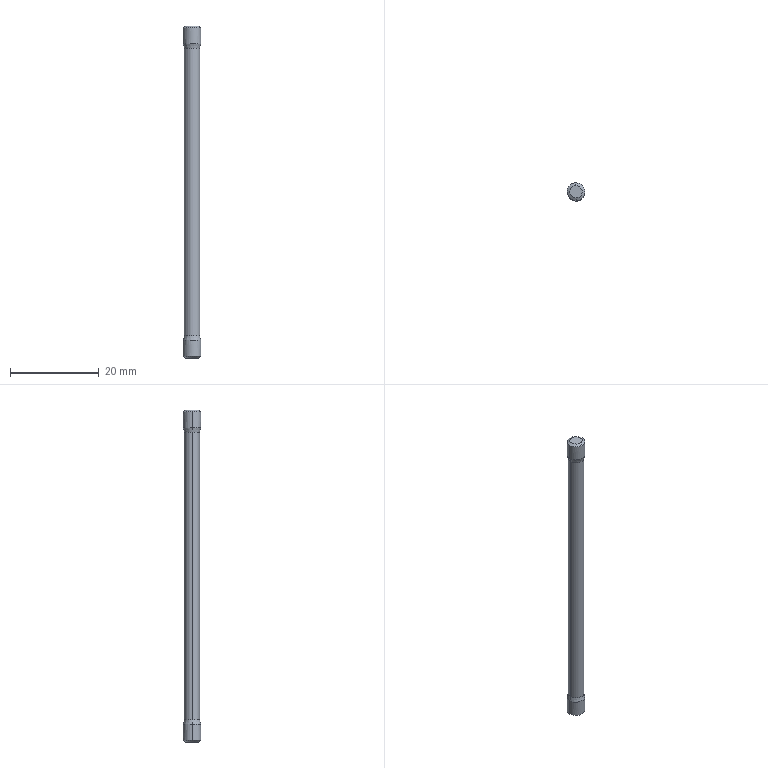Component | SolidWorks | GB_T901-1988EqualLengthDoubleEndStudGradeBM4x75-1 | 1 solid | 16 faces | box 4 x 4 x 75 mm | volume 733 mm3 | cone 8 | cylinder 6 | plane 2 | commonest cylinder face diameters 4 x4 3.464 x2
build123d program:
from build123d import *


with BuildPart() as part:
    # Sketch1 → Base-Revolve (revolve)
    with BuildSketch(Plane.XY, mode=Mode.PRIVATE) as base_revolve_sk:
        Polygon((-37.5, 2), (-33.5, 2), (-32.52, 1.732), (0, 1.732), (0, 0), (-37.5, 0), align=None)
    revolve(base_revolve_sk.sketch.rotate(Axis((-37.5, 0, 0), (1, 0, 0)), 180), axis=Axis((-37.5, 0, 0), (1, 0, 0)))

    # Sketch2 → Thread Cut (revolve, cut)
    with BuildSketch(Plane.XY, mode=Mode.PRIVATE) as thread_cut_sk:
        Polygon((-37.85, 2), (-37.15, 2), (-37.5, 1.394), align=None)
    revolve(thread_cut_sk.sketch.rotate(Axis((-26.952, 0, 0), (1, 0, 0)), 180), axis=Axis((-26.952, 0, 0), (1, 0, 0)), mode=Mode.SUBTRACT)

    # Mirror All1: part across plane


with BuildPart() as part_1:
    add(part.part)
    add(part.part.mirror(Plane(origin=(0, 1.732, 0), x_dir=(0, 0, 1), z_dir=(-1, 0, 0))))


solid = part_1.part

# Placed as in the assembly
solid = solid.moved(Location((18.125, -13.646, 22.463), (0, 90, 0)))
STEP:
#1=CARTESIAN_POINT('',(0.7155,-0.5921,2.361));
#2=VERTEX_POINT('',#1);
#3=CARTESIAN_POINT('',(0.7117,-0.4824,2.361));
#4=VERTEX_POINT('',#3);
#5=CARTESIAN_POINT('',(0.7136,-0.5373,2.361));
#6=DIRECTION('',(0.,0.,-1.));
#7=DIRECTION('',(-0.0348,0.9994,0.));
#8=AXIS2_PLACEMENT_3D('',#5,#6,#7);
#9=CIRCLE('',#8,0.05487);
#10=EDGE_CURVE('',#2,#4,#9,.T.);
#11=ORIENTED_EDGE('',*,*,#10,.T.);
#12=CARTESIAN_POINT('',(0.7108,-0.4586,2.347));
#13=VERTEX_POINT('',#12);
#14=CARTESIAN_POINT('',(0.7117,-0.4824,2.361));
#15=DIRECTION('',(-0.03014,0.8655,-0.5));
#16=VECTOR('',#15,39.37);
#17=LINE('',#14,#16);
#18=EDGE_CURVE('',#4,#13,#17,.T.);
#19=ORIENTED_EDGE('',*,*,#18,.T.);
#20=CARTESIAN_POINT('',(0.6349,-0.54,2.347));
#21=VERTEX_POINT('',#20);
#22=CARTESIAN_POINT('',(0.7136,-0.5373,2.347));
#23=DIRECTION('',(0.,0.,-1.));
#24=DIRECTION('',(-0.0348,0.9994,0.));
#25=AXIS2_PLACEMENT_3D('',#22,#23,#24);
#26=CIRCLE('',#25,0.07874);
#27=EDGE_CURVE('',#21,#13,#26,.T.);
#28=ORIENTED_EDGE('',*,*,#27,.F.);
#29=CARTESIAN_POINT('',(0.7163,-0.616,2.347));
#30=VERTEX_POINT('',#29);
#31=CARTESIAN_POINT('',(0.7136,-0.5373,2.347));
#32=DIRECTION('',(0.,0.,-1.));
#33=DIRECTION('',(-0.0348,0.9994,0.));
#34=AXIS2_PLACEMENT_3D('',#31,#32,#33);
#35=CIRCLE('',#34,0.07874);
#36=EDGE_CURVE('',#30,#21,#35,.T.);
#37=ORIENTED_EDGE('',*,*,#36,.F.);
#38=CARTESIAN_POINT('',(0.7155,-0.5921,2.361));
#39=DIRECTION('',(0.03014,-0.8655,-0.5));
#40=VECTOR('',#39,39.37);
#41=LINE('',#38,#40);
#42=EDGE_CURVE('',#2,#30,#41,.T.);
#43=ORIENTED_EDGE('',*,*,#42,.F.);
#44=EDGE_LOOP('',(#11,#19,#28,#37,#43));
#45=FACE_OUTER_BOUND('',#44,.T.);
#46=CARTESIAN_POINT('',(0.7136,-0.5373,2.361));
#47=DIRECTION('',(0.,0.,-1.));
#48=DIRECTION('',(0.0348,-0.9994,0.));
#49=AXIS2_PLACEMENT_3D('',#46,#47,#48);
#50=CONICAL_SURFACE('',#49,0.05487,1.047);
#51=ADVANCED_FACE('',(#45),#50,.T.);
#52=CARTESIAN_POINT('',(0.7817,-0.5349,2.165));
#53=VERTEX_POINT('',#52);
#54=CARTESIAN_POINT('',(0.6454,-0.5396,2.165));
#55=VERTEX_POINT('',#54);
#56=CARTESIAN_POINT('',(0.7136,-0.5373,2.165));
#57=DIRECTION('',(0.,0.,-1.));
#58=DIRECTION('',(-0.9994,-0.0348,0.));
#59=AXIS2_PLACEMENT_3D('',#56,#57,#58);
#60=CIRCLE('',#59,0.06819);
#61=EDGE_CURVE('',#53,#55,#60,.T.);
#62=ORIENTED_EDGE('',*,*,#61,.F.);
#63=CARTESIAN_POINT('',(0.7923,-0.5345,2.203));
#64=VERTEX_POINT('',#63);
#65=CARTESIAN_POINT('',(0.7817,-0.5349,2.165));
#66=DIRECTION('',(0.2636,0.00918,0.9646));
#67=VECTOR('',#66,39.37);
#68=LINE('',#65,#67);
#69=EDGE_CURVE('',#53,#64,#68,.T.);
#70=ORIENTED_EDGE('',*,*,#69,.T.);
#71=CARTESIAN_POINT('',(0.6349,-0.54,2.203));
#72=VERTEX_POINT('',#71);
#73=CARTESIAN_POINT('',(0.7136,-0.5373,2.203));
#74=DIRECTION('',(0.,0.,-1.));
#75=DIRECTION('',(-0.9994,-0.0348,0.));
#76=AXIS2_PLACEMENT_3D('',#73,#74,#75);
#77=CIRCLE('',#76,0.07874);
#78=EDGE_CURVE('',#64,#72,#77,.T.);
#79=ORIENTED_EDGE('',*,*,#78,.T.);
#80=CARTESIAN_POINT('',(0.6454,-0.5396,2.165));
#81=DIRECTION('',(-0.2636,-0.00918,0.9646));
#82=VECTOR('',#81,39.37);
#83=LINE('',#80,#82);
#84=EDGE_CURVE('',#55,#72,#83,.T.);
#85=ORIENTED_EDGE('',*,*,#84,.F.);
#86=EDGE_LOOP('',(#62,#70,#79,#85));
#87=FACE_OUTER_BOUND('',#86,.T.);
#88=CARTESIAN_POINT('',(0.7136,-0.5373,2.165));
#89=DIRECTION('',(-0.,-0.,1.));
#90=DIRECTION('',(-0.9994,-0.0348,0.));
#91=AXIS2_PLACEMENT_3D('',#88,#89,#90);
#92=CONICAL_SURFACE('',#91,0.06819,0.2669);
#93=ADVANCED_FACE('',(#87),#92,.T.);
#94=ORIENTED_EDGE('',*,*,#78,.F.);
#95=CARTESIAN_POINT('',(0.7923,-0.5345,2.347));
#96=VERTEX_POINT('',#95);
#97=CARTESIAN_POINT('',(0.7923,-0.5345,2.361));
#98=DIRECTION('',(-0.,-0.,1.));
#99=VECTOR('',#98,39.37);
#100=LINE('',#97,#99);
#101=EDGE_CURVE('',#64,#96,#100,.T.);
#102=ORIENTED_EDGE('',*,*,#101,.T.);
#103=CARTESIAN_POINT('',(0.7136,-0.5373,2.347));
#104=DIRECTION('',(0.,0.,-1.));
#105=DIRECTION('',(-0.0348,0.9994,0.));
#106=AXIS2_PLACEMENT_3D('',#103,#104,#105);
#107=CIRCLE('',#106,0.07874);
#108=EDGE_CURVE('',#96,#30,#107,.T.);
#109=ORIENTED_EDGE('',*,*,#108,.T.);
#110=ORIENTED_EDGE('',*,*,#36,.T.);
#111=CARTESIAN_POINT('',(0.6349,-0.54,2.361));
#112=DIRECTION('',(-0.,-0.,1.));
#113=VECTOR('',#112,39.37);
#114=LINE('',#111,#113);
#115=EDGE_CURVE('',#72,#21,#114,.T.);
#116=ORIENTED_EDGE('',*,*,#115,.F.);
#117=EDGE_LOOP('',(#94,#102,#109,#110,#116));
#118=FACE_OUTER_BOUND('',#117,.T.);
#119=CARTESIAN_POINT('',(0.7136,-0.5373,2.361));
#120=DIRECTION('',(-0.,-0.,1.));
#121=DIRECTION('',(-0.9994,-0.0348,0.));
#122=AXIS2_PLACEMENT_3D('',#119,#120,#121);
#123=CYLINDRICAL_SURFACE('',#122,0.07874);
#124=ADVANCED_FACE('',(#118),#123,.T.);
#125=CARTESIAN_POINT('',(0.7117,-0.4824,-0.592));
#126=VERTEX_POINT('',#125);
#127=CARTESIAN_POINT('',(0.7155,-0.5921,-0.592));
#128=VERTEX_POINT('',#127);
#129=CARTESIAN_POINT('',(0.7136,-0.5373,-0.592));
#130=DIRECTION('',(0.,0.,-1.));
#131=DIRECTION('',(-0.0348,0.9994,0.));
#132=AXIS2_PLACEMENT_3D('',#129,#130,#131);
#133=CIRCLE('',#132,0.05487);
#134=EDGE_CURVE('',#126,#128,#133,.T.);
#135=ORIENTED_EDGE('',*,*,#134,.F.);
#136=CARTESIAN_POINT('',(0.7108,-0.4586,-0.5782));
#137=VERTEX_POINT('',#136);
#138=CARTESIAN_POINT('',(0.7117,-0.4824,-0.592));
#139=DIRECTION('',(-0.03014,0.8655,0.5));
#140=VECTOR('',#139,39.37);
#141=LINE('',#138,#140);
#142=EDGE_CURVE('',#126,#137,#141,.T.);
#143=ORIENTED_EDGE('',*,*,#142,.T.);
#144=CARTESIAN_POINT('',(0.7923,-0.5345,-0.5782));
#145=VERTEX_POINT('',#144);
#146=CARTESIAN_POINT('',(0.7136,-0.5373,-0.5782));
#147=DIRECTION('',(0.,0.,-1.));
#148=DIRECTION('',(-0.0348,0.9994,0.));
#149=AXIS2_PLACEMENT_3D('',#146,#147,#148);
#150=CIRCLE('',#149,0.07874);
#151=EDGE_CURVE('',#137,#145,#150,.T.);
#152=ORIENTED_EDGE('',*,*,#151,.T.);
#153=CARTESIAN_POINT('',(0.7163,-0.616,-0.5782));
#154=VERTEX_POINT('',#153);
#155=CARTESIAN_POINT('',(0.7136,-0.5373,-0.5782));
#156=DIRECTION('',(0.,0.,-1.));
#157=DIRECTION('',(-0.0348,0.9994,0.));
#158=AXIS2_PLACEMENT_3D('',#155,#156,#157);
#159=CIRCLE('',#158,0.07874);
#160=EDGE_CURVE('',#145,#154,#159,.T.);
#161=ORIENTED_EDGE('',*,*,#160,.T.);
#162=CARTESIAN_POINT('',(0.7155,-0.5921,-0.592));
#163=DIRECTION('',(0.03014,-0.8655,0.5));
#164=VECTOR('',#163,39.37);
#165=LINE('',#162,#164);
#166=EDGE_CURVE('',#128,#154,#165,.T.);
#167=ORIENTED_EDGE('',*,*,#166,.F.);
#168=EDGE_LOOP('',(#135,#143,#152,#161,#167));
#169=FACE_OUTER_BOUND('',#168,.T.);
#170=CARTESIAN_POINT('',(0.7136,-0.5373,-0.592));
#171=DIRECTION('',(-0.,-0.,1.));
#172=DIRECTION('',(0.0348,-0.9994,0.));
#173=AXIS2_PLACEMENT_3D('',#170,#171,#172);
#174=CONICAL_SURFACE('',#173,0.05487,1.047);
#175=ADVANCED_FACE('',(#169),#174,.T.);
#176=CARTESIAN_POINT('',(0.6454,-0.5396,-0.3959));
#177=VERTEX_POINT('',#176);
#178=CARTESIAN_POINT('',(0.7817,-0.5349,-0.3959));
#179=VERTEX_POINT('',#178);
#180=CARTESIAN_POINT('',(0.7136,-0.5373,-0.3959));
#181=DIRECTION('',(0.,0.,-1.));
#182=DIRECTION('',(-0.9994,-0.0348,0.));
#183=AXIS2_PLACEMENT_3D('',#180,#181,#182);
#184=CIRCLE('',#183,0.06819);
#185=EDGE_CURVE('',#177,#179,#184,.T.);
#186=ORIENTED_EDGE('',*,*,#185,.T.);
#187=CARTESIAN_POINT('',(0.7923,-0.5345,-0.4345));
#188=VERTEX_POINT('',#187);
#189=CARTESIAN_POINT('',(0.7817,-0.5349,-0.3959));
#190=DIRECTION('',(0.2636,0.00918,-0.9646));
#191=VECTOR('',#190,39.37);
#192=LINE('',#189,#191);
#193=EDGE_CURVE('',#179,#188,#192,.T.);
#194=ORIENTED_EDGE('',*,*,#193,.T.);
#195=CARTESIAN_POINT('',(0.6349,-0.54,-0.4345));
#196=VERTEX_POINT('',#195);
#197=CARTESIAN_POINT('',(0.7136,-0.5373,-0.4345));
#198=DIRECTION('',(0.,0.,-1.));
#199=DIRECTION('',(-0.9994,-0.0348,0.));
#200=AXIS2_PLACEMENT_3D('',#197,#198,#199);
#201=CIRCLE('',#200,0.07874);
#202=EDGE_CURVE('',#196,#188,#201,.T.);
#203=ORIENTED_EDGE('',*,*,#202,.F.);
#204=CARTESIAN_POINT('',(0.6454,-0.5396,-0.3959));
#205=DIRECTION('',(-0.2636,-0.00918,-0.9646));
#206=VECTOR('',#205,39.37);
#207=LINE('',#204,#206);
#208=EDGE_CURVE('',#177,#196,#207,.T.);
#209=ORIENTED_EDGE('',*,*,#208,.F.);
#210=EDGE_LOOP('',(#186,#194,#203,#209));
#211=FACE_OUTER_BOUND('',#210,.T.);
#212=CARTESIAN_POINT('',(0.7136,-0.5373,-0.3959));
#213=DIRECTION('',(0.,0.,-1.));
#214=DIRECTION('',(-0.9994,-0.0348,0.));
#215=AXIS2_PLACEMENT_3D('',#212,#213,#214);
#216=CONICAL_SURFACE('',#215,0.06819,0.2669);
#217=ADVANCED_FACE('',(#211),#216,.T.);
#218=CARTESIAN_POINT('',(0.7136,-0.5373,2.165));
#219=DIRECTION('',(0.,0.,-1.));
#220=DIRECTION('',(-0.9994,-0.0348,0.));
#221=AXIS2_PLACEMENT_3D('',#218,#219,#220);
#222=CIRCLE('',#221,0.06819);
#223=EDGE_CURVE('',#55,#53,#222,.T.);
#224=ORIENTED_EDGE('',*,*,#223,.T.);
#225=CARTESIAN_POINT('',(0.7817,-0.5349,-0.592));
#226=DIRECTION('',(0.,0.,-1.));
#227=VECTOR('',#226,39.37);
#228=LINE('',#225,#227);
#229=EDGE_CURVE('',#53,#179,#228,.T.);
#230=ORIENTED_EDGE('',*,*,#229,.T.);
#231=ORIENTED_EDGE('',*,*,#185,.F.);
#232=CARTESIAN_POINT('',(0.6454,-0.5396,-0.592));
#233=DIRECTION('',(0.,0.,-1.));
#234=VECTOR('',#233,39.37);
#235=LINE('',#232,#234);
#236=EDGE_CURVE('',#55,#177,#235,.T.);
#237=ORIENTED_EDGE('',*,*,#236,.F.);
#238=EDGE_LOOP('',(#224,#230,#231,#237));
#239=FACE_OUTER_BOUND('',#238,.T.);
#240=CARTESIAN_POINT('',(0.7136,-0.5373,-0.592));
#241=DIRECTION('',(0.,0.,-1.));
#242=DIRECTION('',(-0.9994,-0.0348,0.));
#243=AXIS2_PLACEMENT_3D('',#240,#241,#242);
#244=CYLINDRICAL_SURFACE('',#243,0.06819);
#245=ADVANCED_FACE('',(#239),#244,.T.);
#246=ORIENTED_EDGE('',*,*,#202,.T.);
#247=CARTESIAN_POINT('',(0.7923,-0.5345,-0.592));
#248=DIRECTION('',(0.,0.,-1.));
#249=VECTOR('',#248,39.37);
#250=LINE('',#247,#249);
#251=EDGE_CURVE('',#188,#145,#250,.T.);
#252=ORIENTED_EDGE('',*,*,#251,.T.);
#253=ORIENTED_EDGE('',*,*,#151,.F.);
#254=CARTESIAN_POINT('',(0.6349,-0.54,-0.5782));
#255=VERTEX_POINT('',#254);
#256=CARTESIAN_POINT('',(0.7136,-0.5373,-0.5782));
#257=DIRECTION('',(0.,0.,-1.));
#258=DIRECTION('',(-0.0348,0.9994,0.));
#259=AXIS2_PLACEMENT_3D('',#256,#257,#258);
#260=CIRCLE('',#259,0.07874);
#261=EDGE_CURVE('',#255,#137,#260,.T.);
#262=ORIENTED_EDGE('',*,*,#261,.F.);
#263=CARTESIAN_POINT('',(0.6349,-0.54,-0.592));
#264=DIRECTION('',(0.,0.,-1.));
#265=VECTOR('',#264,39.37);
#266=LINE('',#263,#265);
#267=EDGE_CURVE('',#196,#255,#266,.T.);
#268=ORIENTED_EDGE('',*,*,#267,.F.);
#269=EDGE_LOOP('',(#246,#252,#253,#262,#268));
#270=FACE_OUTER_BOUND('',#269,.T.);
#271=CARTESIAN_POINT('',(0.7136,-0.5373,-0.592));
#272=DIRECTION('',(0.,0.,-1.));
#273=DIRECTION('',(-0.9994,-0.0348,0.));
#274=AXIS2_PLACEMENT_3D('',#271,#272,#273);
#275=CYLINDRICAL_SURFACE('',#274,0.07874);
#276=ADVANCED_FACE('',(#270),#275,.T.);
#277=ORIENTED_EDGE('',*,*,#251,.F.);
#278=CARTESIAN_POINT('',(0.7136,-0.5373,-0.4345));
#279=DIRECTION('',(0.,0.,-1.));
#280=DIRECTION('',(-0.9994,-0.0348,0.));
#281=AXIS2_PLACEMENT_3D('',#278,#279,#280);
#282=CIRCLE('',#281,0.07874);
#283=EDGE_CURVE('',#188,#196,#282,.T.);
#284=ORIENTED_EDGE('',*,*,#283,.T.);
#285=ORIENTED_EDGE('',*,*,#267,.T.);
#286=CARTESIAN_POINT('',(0.7136,-0.5373,-0.5782));
#287=DIRECTION('',(0.,0.,-1.));
#288=DIRECTION('',(-0.0348,0.9994,0.));
#289=AXIS2_PLACEMENT_3D('',#286,#287,#288);
#290=CIRCLE('',#289,0.07874);
#291=EDGE_CURVE('',#154,#255,#290,.T.);
#292=ORIENTED_EDGE('',*,*,#291,.F.);
#293=ORIENTED_EDGE('',*,*,#160,.F.);
#294=EDGE_LOOP('',(#277,#284,#285,#292,#293));
#295=FACE_OUTER_BOUND('',#294,.T.);
#296=CARTESIAN_POINT('',(0.7136,-0.5373,-0.592));
#297=DIRECTION('',(0.,0.,-1.));
#298=DIRECTION('',(-0.9994,-0.0348,0.));
#299=AXIS2_PLACEMENT_3D('',#296,#297,#298);
#300=CYLINDRICAL_SURFACE('',#299,0.07874);
#301=ADVANCED_FACE('',(#295),#300,.T.);
#302=ORIENTED_EDGE('',*,*,#229,.F.);
#303=ORIENTED_EDGE('',*,*,#61,.T.);
#304=ORIENTED_EDGE('',*,*,#236,.T.);
#305=CARTESIAN_POINT('',(0.7136,-0.5373,-0.3959));
#306=DIRECTION('',(0.,0.,-1.));
#307=DIRECTION('',(-0.9994,-0.0348,0.));
#308=AXIS2_PLACEMENT_3D('',#305,#306,#307);
#309=CIRCLE('',#308,0.06819);
#310=EDGE_CURVE('',#179,#177,#309,.T.);
#311=ORIENTED_EDGE('',*,*,#310,.F.);
#312=EDGE_LOOP('',(#302,#303,#304,#311));
#313=FACE_OUTER_BOUND('',#312,.T.);
#314=CARTESIAN_POINT('',(0.7136,-0.5373,-0.592));
#315=DIRECTION('',(0.,0.,-1.));
#316=DIRECTION('',(-0.9994,-0.0348,0.));
#317=AXIS2_PLACEMENT_3D('',#314,#315,#316);
#318=CYLINDRICAL_SURFACE('',#317,0.06819);
#319=ADVANCED_FACE('',(#313),#318,.T.);
#320=ORIENTED_EDGE('',*,*,#193,.F.);
#321=ORIENTED_EDGE('',*,*,#310,.T.);
#322=ORIENTED_EDGE('',*,*,#208,.T.);
#323=ORIENTED_EDGE('',*,*,#283,.F.);
#324=EDGE_LOOP('',(#320,#321,#322,#323));
#325=FACE_OUTER_BOUND('',#324,.T.);
#326=CARTESIAN_POINT('',(0.7136,-0.5373,-0.3959));
#327=DIRECTION('',(0.,0.,-1.));
#328=DIRECTION('',(-0.9994,-0.0348,0.));
#329=AXIS2_PLACEMENT_3D('',#326,#327,#328);
#330=CONICAL_SURFACE('',#329,0.06819,0.2669);
#331=ADVANCED_FACE('',(#325),#330,.T.);
#332=ORIENTED_EDGE('',*,*,#142,.F.);
#333=CARTESIAN_POINT('',(0.7136,-0.5373,-0.592));
#334=DIRECTION('',(0.,0.,-1.));
#335=DIRECTION('',(-0.0348,0.9994,0.));
#336=AXIS2_PLACEMENT_3D('',#333,#334,#335);
#337=CIRCLE('',#336,0.05487);
#338=EDGE_CURVE('',#128,#126,#337,.T.);
#339=ORIENTED_EDGE('',*,*,#338,.F.);
#340=ORIENTED_EDGE('',*,*,#166,.T.);
#341=ORIENTED_EDGE('',*,*,#291,.T.);
#342=ORIENTED_EDGE('',*,*,#261,.T.);
#343=EDGE_LOOP('',(#332,#339,#340,#341,#342));
#344=FACE_OUTER_BOUND('',#343,.T.);
#345=CARTESIAN_POINT('',(0.7136,-0.5373,-0.592));
#346=DIRECTION('',(-0.,-0.,1.));
#347=DIRECTION('',(0.0348,-0.9994,0.));
#348=AXIS2_PLACEMENT_3D('',#345,#346,#347);
#349=CONICAL_SURFACE('',#348,0.05487,1.047);
#350=ADVANCED_FACE('',(#344),#349,.T.);
#351=ORIENTED_EDGE('',*,*,#338,.T.);
#352=ORIENTED_EDGE('',*,*,#134,.T.);
#353=EDGE_LOOP('',(#351,#352));
#354=FACE_OUTER_BOUND('',#353,.T.);
#355=CARTESIAN_POINT('',(0.7923,-0.5345,-0.592));
#356=DIRECTION('',(-0.,-0.,1.));
#357=DIRECTION('',(0.9994,0.0348,0.));
#358=AXIS2_PLACEMENT_3D('',#355,#356,#357);
#359=PLANE('',#358);
#360=ADVANCED_FACE('',(#354),#359,.F.);
#361=ORIENTED_EDGE('',*,*,#101,.F.);
#362=CARTESIAN_POINT('',(0.7136,-0.5373,2.203));
#363=DIRECTION('',(0.,0.,-1.));
#364=DIRECTION('',(-0.9994,-0.0348,0.));
#365=AXIS2_PLACEMENT_3D('',#362,#363,#364);
#366=CIRCLE('',#365,0.07874);
#367=EDGE_CURVE('',#72,#64,#366,.T.);
#368=ORIENTED_EDGE('',*,*,#367,.F.);
#369=ORIENTED_EDGE('',*,*,#115,.T.);
#370=ORIENTED_EDGE('',*,*,#27,.T.);
#371=CARTESIAN_POINT('',(0.7136,-0.5373,2.347));
#372=DIRECTION('',(0.,0.,-1.));
#373=DIRECTION('',(-0.0348,0.9994,0.));
#374=AXIS2_PLACEMENT_3D('',#371,#372,#373);
#375=CIRCLE('',#374,0.07874);
#376=EDGE_CURVE('',#13,#96,#375,.T.);
#377=ORIENTED_EDGE('',*,*,#376,.T.);
#378=EDGE_LOOP('',(#361,#368,#369,#370,#377));
#379=FACE_OUTER_BOUND('',#378,.T.);
#380=CARTESIAN_POINT('',(0.7136,-0.5373,2.361));
#381=DIRECTION('',(-0.,-0.,1.));
#382=DIRECTION('',(-0.9994,-0.0348,0.));
#383=AXIS2_PLACEMENT_3D('',#380,#381,#382);
#384=CYLINDRICAL_SURFACE('',#383,0.07874);
#385=ADVANCED_FACE('',(#379),#384,.T.);
#386=ORIENTED_EDGE('',*,*,#69,.F.);
#387=ORIENTED_EDGE('',*,*,#223,.F.);
#388=ORIENTED_EDGE('',*,*,#84,.T.);
#389=ORIENTED_EDGE('',*,*,#367,.T.);
#390=EDGE_LOOP('',(#386,#387,#388,#389));
#391=FACE_OUTER_BOUND('',#390,.T.);
#392=CARTESIAN_POINT('',(0.7136,-0.5373,2.165));
#393=DIRECTION('',(-0.,-0.,1.));
#394=DIRECTION('',(-0.9994,-0.0348,0.));
#395=AXIS2_PLACEMENT_3D('',#392,#393,#394);
#396=CONICAL_SURFACE('',#395,0.06819,0.2669);
#397=ADVANCED_FACE('',(#391),#396,.T.);
#398=ORIENTED_EDGE('',*,*,#18,.F.);
#399=CARTESIAN_POINT('',(0.7136,-0.5373,2.361));
#400=DIRECTION('',(0.,0.,-1.));
#401=DIRECTION('',(-0.0348,0.9994,0.));
#402=AXIS2_PLACEMENT_3D('',#399,#400,#401);
#403=CIRCLE('',#402,0.05487);
#404=EDGE_CURVE('',#4,#2,#403,.T.);
#405=ORIENTED_EDGE('',*,*,#404,.T.);
#406=ORIENTED_EDGE('',*,*,#42,.T.);
#407=ORIENTED_EDGE('',*,*,#108,.F.);
#408=ORIENTED_EDGE('',*,*,#376,.F.);
#409=EDGE_LOOP('',(#398,#405,#406,#407,#408));
#410=FACE_OUTER_BOUND('',#409,.T.);
#411=CARTESIAN_POINT('',(0.7136,-0.5373,2.361));
#412=DIRECTION('',(0.,0.,-1.));
#413=DIRECTION('',(0.0348,-0.9994,0.));
#414=AXIS2_PLACEMENT_3D('',#411,#412,#413);
#415=CONICAL_SURFACE('',#414,0.05487,1.047);
#416=ADVANCED_FACE('',(#410),#415,.T.);
#417=ORIENTED_EDGE('',*,*,#10,.F.);
#418=ORIENTED_EDGE('',*,*,#404,.F.);
#419=EDGE_LOOP('',(#417,#418));
#420=FACE_OUTER_BOUND('',#419,.T.);
#421=CARTESIAN_POINT('',(0.7923,-0.5345,2.361));
#422=DIRECTION('',(0.,0.,-1.));
#423=DIRECTION('',(0.9994,0.0348,0.));
#424=AXIS2_PLACEMENT_3D('',#421,#422,#423);
#425=PLANE('',#424);
#426=ADVANCED_FACE('',(#420),#425,.F.);
#427=CLOSED_SHELL('',(#51,#93,#124,#175,#217,#245,#276,#301,#319,#331,#350,#360,#385,#397,#416,#426));
#428=MANIFOLD_SOLID_BREP('',#427);
#429=CARTESIAN_POINT('',(0.,0.,0.));
#430=DIRECTION('',(0.,0.,1.));
#431=DIRECTION('',(1.,0.,0.));
#432=AXIS2_PLACEMENT_3D('',#429,#430,#431);
#433=(LENGTH_UNIT()NAMED_UNIT(*)SI_UNIT($,.METRE.));
#434=LENGTH_MEASURE_WITH_UNIT(LENGTH_MEASURE(0.0254),#433);
#435=DIMENSIONAL_EXPONENTS(1.,0.,0.,0.,0.,0.,0.);
#436=(CONVERSION_BASED_UNIT('',#434)LENGTH_UNIT()NAMED_UNIT(#435));
#437=UNCERTAINTY_MEASURE_WITH_UNIT(LENGTH_MEASURE(0.00001),#436,'','');
#438=(NAMED_UNIT(*)PLANE_ANGLE_UNIT()SI_UNIT($,.RADIAN.));
#439=(NAMED_UNIT(*)SI_UNIT($,.STERADIAN.)SOLID_ANGLE_UNIT());
#440=(GEOMETRIC_REPRESENTATION_CONTEXT(3)GLOBAL_UNCERTAINTY_ASSIGNED_CONTEXT((#437))GLOBAL_UNIT_ASSIGNED_CONTEXT((#436,#438,#439))REPRESENTATION_CONTEXT('',''));
#441=ADVANCED_BREP_SHAPE_REPRESENTATION('',(#428,#432),#440);
#442=COLOUR_RGB('',0.7922,0.8196,0.9333);
#443=FILL_AREA_STYLE_COLOUR('',#442);
#444=FILL_AREA_STYLE('',(#443));
#445=SURFACE_STYLE_FILL_AREA(#444);
#446=SURFACE_SIDE_STYLE('',(#445));
#447=SURFACE_STYLE_USAGE(.BOTH.,#446);
#448=PRESENTATION_STYLE_ASSIGNMENT((#447));
#449=STYLED_ITEM('',(#448),#428);
#450=(LENGTH_UNIT()NAMED_UNIT(*)SI_UNIT($,.METRE.));
#451=LENGTH_MEASURE_WITH_UNIT(LENGTH_MEASURE(0.0254),#450);
#452=DIMENSIONAL_EXPONENTS(1.,0.,0.,0.,0.,0.,0.);
#453=(CONVERSION_BASED_UNIT('',#451)LENGTH_UNIT()NAMED_UNIT(#452));
#454=UNCERTAINTY_MEASURE_WITH_UNIT(LENGTH_MEASURE(0.00001),#453,'','');
#455=(NAMED_UNIT(*)PLANE_ANGLE_UNIT()SI_UNIT($,.RADIAN.));
#456=(NAMED_UNIT(*)SI_UNIT($,.STERADIAN.)SOLID_ANGLE_UNIT());
#457=(GEOMETRIC_REPRESENTATION_CONTEXT(3)GLOBAL_UNCERTAINTY_ASSIGNED_CONTEXT((#454))GLOBAL_UNIT_ASSIGNED_CONTEXT((#453,#455,#456))REPRESENTATION_CONTEXT('',''));
#458=MECHANICAL_DESIGN_GEOMETRIC_PRESENTATION_REPRESENTATION('',(#449),#457);
#459=PRESENTATION_LAYER_ASSIGNMENT('','',(#449));